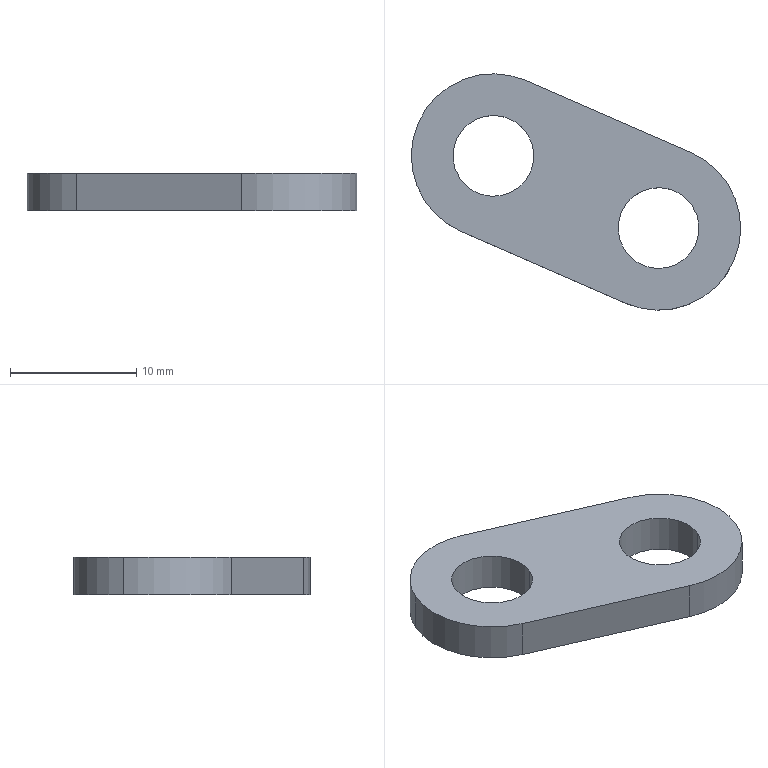Component | SolidWorks | CH-225-D-1_225-D-04-1 | 1 solid | 11 faces | box 26.08 x 18.71 x 3 mm | volume 762 mm3 | cylinder 7 | plane 4 | commonest cylinder face diameters 6.4 x4 13 x3
STEP:
#1=CARTESIAN_POINT('',(1.542,2.996,4.761));
#2=VERTEX_POINT('',#1);
#3=CARTESIAN_POINT('',(1.773,2.895,4.761));
#4=VERTEX_POINT('',#3);
#5=CARTESIAN_POINT('',(1.658,2.945,4.761));
#6=DIRECTION('',(0.,0.,1.));
#7=DIRECTION('',(-0.9164,0.4003,0.));
#8=AXIS2_PLACEMENT_3D('',#5,#6,#7);
#9=CIRCLE('',#8,0.126);
#10=EDGE_CURVE('',#2,#4,#9,.T.);
#11=ORIENTED_EDGE('',*,*,#10,.T.);
#12=CARTESIAN_POINT('',(1.773,2.895,4.643));
#13=VERTEX_POINT('',#12);
#14=CARTESIAN_POINT('',(1.773,2.895,4.761));
#15=DIRECTION('',(0.,0.,-1.));
#16=VECTOR('',#15,39.37);
#17=LINE('',#14,#16);
#18=EDGE_CURVE('',#4,#13,#17,.T.);
#19=ORIENTED_EDGE('',*,*,#18,.T.);
#20=CARTESIAN_POINT('',(1.542,2.996,4.643));
#21=VERTEX_POINT('',#20);
#22=CARTESIAN_POINT('',(1.658,2.945,4.643));
#23=DIRECTION('',(0.,0.,-1.));
#24=DIRECTION('',(-0.9164,0.4003,0.));
#25=AXIS2_PLACEMENT_3D('',#22,#23,#24);
#26=CIRCLE('',#25,0.126);
#27=EDGE_CURVE('',#13,#21,#26,.T.);
#28=ORIENTED_EDGE('',*,*,#27,.T.);
#29=CARTESIAN_POINT('',(1.542,2.996,4.761));
#30=DIRECTION('',(0.,0.,-1.));
#31=VECTOR('',#30,39.37);
#32=LINE('',#29,#31);
#33=EDGE_CURVE('',#2,#21,#32,.T.);
#34=ORIENTED_EDGE('',*,*,#33,.F.);
#35=EDGE_LOOP('',(#11,#19,#28,#34));
#36=FACE_OUTER_BOUND('',#35,.T.);
#37=CARTESIAN_POINT('',(1.658,2.945,4.761));
#38=DIRECTION('',(0.,0.,-1.));
#39=DIRECTION('',(-0.9164,0.4003,0.));
#40=AXIS2_PLACEMENT_3D('',#37,#38,#39);
#41=CYLINDRICAL_SURFACE('',#40,0.126);
#42=ADVANCED_FACE('',(#36),#41,.F.);
#43=CARTESIAN_POINT('',(2.288,2.67,4.761));
#44=VERTEX_POINT('',#43);
#45=CARTESIAN_POINT('',(2.057,2.771,4.761));
#46=VERTEX_POINT('',#45);
#47=CARTESIAN_POINT('',(2.172,2.721,4.761));
#48=DIRECTION('',(0.,0.,-1.));
#49=DIRECTION('',(-0.9164,0.4003,0.));
#50=AXIS2_PLACEMENT_3D('',#47,#48,#49);
#51=CIRCLE('',#50,0.126);
#52=EDGE_CURVE('',#44,#46,#51,.T.);
#53=ORIENTED_EDGE('',*,*,#52,.F.);
#54=CARTESIAN_POINT('',(2.288,2.67,4.643));
#55=VERTEX_POINT('',#54);
#56=CARTESIAN_POINT('',(2.288,2.67,4.761));
#57=DIRECTION('',(0.,0.,-1.));
#58=VECTOR('',#57,39.37);
#59=LINE('',#56,#58);
#60=EDGE_CURVE('',#44,#55,#59,.T.);
#61=ORIENTED_EDGE('',*,*,#60,.T.);
#62=CARTESIAN_POINT('',(2.057,2.771,4.643));
#63=VERTEX_POINT('',#62);
#64=CARTESIAN_POINT('',(2.172,2.721,4.643));
#65=DIRECTION('',(0.,0.,-1.));
#66=DIRECTION('',(-0.9164,0.4003,0.));
#67=AXIS2_PLACEMENT_3D('',#64,#65,#66);
#68=CIRCLE('',#67,0.126);
#69=EDGE_CURVE('',#55,#63,#68,.T.);
#70=ORIENTED_EDGE('',*,*,#69,.T.);
#71=CARTESIAN_POINT('',(2.057,2.771,4.761));
#72=DIRECTION('',(0.,0.,-1.));
#73=VECTOR('',#72,39.37);
#74=LINE('',#71,#73);
#75=EDGE_CURVE('',#46,#63,#74,.T.);
#76=ORIENTED_EDGE('',*,*,#75,.F.);
#77=EDGE_LOOP('',(#53,#61,#70,#76));
#78=FACE_OUTER_BOUND('',#77,.T.);
#79=CARTESIAN_POINT('',(2.172,2.721,4.761));
#80=DIRECTION('',(0.,0.,-1.));
#81=DIRECTION('',(-0.9164,0.4003,0.));
#82=AXIS2_PLACEMENT_3D('',#79,#80,#81);
#83=CYLINDRICAL_SURFACE('',#82,0.126);
#84=ADVANCED_FACE('',(#78),#83,.F.);
#85=CARTESIAN_POINT('',(1.423,3.048,4.761));
#86=VERTEX_POINT('',#85);
#87=CARTESIAN_POINT('',(1.555,2.711,4.761));
#88=VERTEX_POINT('',#87);
#89=CARTESIAN_POINT('',(1.658,2.945,4.761));
#90=DIRECTION('',(0.,0.,1.));
#91=DIRECTION('',(-0.9164,0.4003,0.));
#92=AXIS2_PLACEMENT_3D('',#89,#90,#91);
#93=CIRCLE('',#92,0.2559);
#94=EDGE_CURVE('',#86,#88,#93,.T.);
#95=ORIENTED_EDGE('',*,*,#94,.F.);
#96=CARTESIAN_POINT('',(1.423,3.048,4.643));
#97=VERTEX_POINT('',#96);
#98=CARTESIAN_POINT('',(1.423,3.048,4.761));
#99=DIRECTION('',(0.,0.,-1.));
#100=VECTOR('',#99,39.37);
#101=LINE('',#98,#100);
#102=EDGE_CURVE('',#86,#97,#101,.T.);
#103=ORIENTED_EDGE('',*,*,#102,.T.);
#104=CARTESIAN_POINT('',(1.555,2.711,4.643));
#105=VERTEX_POINT('',#104);
#106=CARTESIAN_POINT('',(1.658,2.945,4.643));
#107=DIRECTION('',(0.,0.,1.));
#108=DIRECTION('',(-0.9164,0.4003,0.));
#109=AXIS2_PLACEMENT_3D('',#106,#107,#108);
#110=CIRCLE('',#109,0.2559);
#111=EDGE_CURVE('',#97,#105,#110,.T.);
#112=ORIENTED_EDGE('',*,*,#111,.T.);
#113=CARTESIAN_POINT('',(1.555,2.711,4.702));
#114=DIRECTION('',(0.,0.,1.));
#115=VECTOR('',#114,39.37);
#116=LINE('',#113,#115);
#117=EDGE_CURVE('',#105,#88,#116,.T.);
#118=ORIENTED_EDGE('',*,*,#117,.T.);
#119=EDGE_LOOP('',(#95,#103,#112,#118));
#120=FACE_OUTER_BOUND('',#119,.T.);
#121=CARTESIAN_POINT('',(1.658,2.945,4.761));
#122=DIRECTION('',(0.,0.,-1.));
#123=DIRECTION('',(-0.9164,0.4003,0.));
#124=AXIS2_PLACEMENT_3D('',#121,#122,#123);
#125=CYLINDRICAL_SURFACE('',#124,0.2559);
#126=ADVANCED_FACE('',(#120),#125,.T.);
#127=ORIENTED_EDGE('',*,*,#18,.F.);
#128=CARTESIAN_POINT('',(1.658,2.945,4.761));
#129=DIRECTION('',(0.,0.,1.));
#130=DIRECTION('',(-0.9164,0.4003,0.));
#131=AXIS2_PLACEMENT_3D('',#128,#129,#130);
#132=CIRCLE('',#131,0.126);
#133=EDGE_CURVE('',#4,#2,#132,.T.);
#134=ORIENTED_EDGE('',*,*,#133,.T.);
#135=ORIENTED_EDGE('',*,*,#33,.T.);
#136=CARTESIAN_POINT('',(1.658,2.945,4.643));
#137=DIRECTION('',(0.,0.,-1.));
#138=DIRECTION('',(-0.9164,0.4003,0.));
#139=AXIS2_PLACEMENT_3D('',#136,#137,#138);
#140=CIRCLE('',#139,0.126);
#141=EDGE_CURVE('',#21,#13,#140,.T.);
#142=ORIENTED_EDGE('',*,*,#141,.T.);
#143=EDGE_LOOP('',(#127,#134,#135,#142));
#144=FACE_OUTER_BOUND('',#143,.T.);
#145=CARTESIAN_POINT('',(1.658,2.945,4.761));
#146=DIRECTION('',(0.,0.,-1.));
#147=DIRECTION('',(-0.9164,0.4003,0.));
#148=AXIS2_PLACEMENT_3D('',#145,#146,#147);
#149=CYLINDRICAL_SURFACE('',#148,0.126);
#150=ADVANCED_FACE('',(#144),#149,.F.);
#151=ORIENTED_EDGE('',*,*,#141,.F.);
#152=ORIENTED_EDGE('',*,*,#27,.F.);
#153=EDGE_LOOP('',(#151,#152));
#154=FACE_BOUND('',#153,.T.);
#155=CARTESIAN_POINT('',(2.172,2.721,4.643));
#156=DIRECTION('',(0.,0.,-1.));
#157=DIRECTION('',(-0.9164,0.4003,0.));
#158=AXIS2_PLACEMENT_3D('',#155,#156,#157);
#159=CIRCLE('',#158,0.126);
#160=EDGE_CURVE('',#63,#55,#159,.T.);
#161=ORIENTED_EDGE('',*,*,#160,.F.);
#162=ORIENTED_EDGE('',*,*,#69,.F.);
#163=EDGE_LOOP('',(#161,#162));
#164=FACE_BOUND('',#163,.T.);
#165=CARTESIAN_POINT('',(2.275,2.955,4.643));
#166=VERTEX_POINT('',#165);
#167=CARTESIAN_POINT('',(1.76,3.18,4.643));
#168=VERTEX_POINT('',#167);
#169=CARTESIAN_POINT('',(2.017,3.067,4.643));
#170=DIRECTION('',(-0.9164,0.4003,0.));
#171=VECTOR('',#170,39.37);
#172=LINE('',#169,#171);
#173=EDGE_CURVE('',#166,#168,#172,.T.);
#174=ORIENTED_EDGE('',*,*,#173,.F.);
#175=CARTESIAN_POINT('',(2.07,2.486,4.643));
#176=VERTEX_POINT('',#175);
#177=CARTESIAN_POINT('',(2.172,2.721,4.643));
#178=DIRECTION('',(0.,0.,1.));
#179=DIRECTION('',(-0.9164,0.4003,0.));
#180=AXIS2_PLACEMENT_3D('',#177,#178,#179);
#181=CIRCLE('',#180,0.2559);
#182=EDGE_CURVE('',#176,#166,#181,.T.);
#183=ORIENTED_EDGE('',*,*,#182,.F.);
#184=CARTESIAN_POINT('',(1.813,2.598,4.643));
#185=DIRECTION('',(0.9164,-0.4003,0.));
#186=VECTOR('',#185,39.37);
#187=LINE('',#184,#186);
#188=EDGE_CURVE('',#105,#176,#187,.T.);
#189=ORIENTED_EDGE('',*,*,#188,.F.);
#190=ORIENTED_EDGE('',*,*,#111,.F.);
#191=CARTESIAN_POINT('',(1.658,2.945,4.643));
#192=DIRECTION('',(0.,0.,1.));
#193=DIRECTION('',(-0.9164,0.4003,0.));
#194=AXIS2_PLACEMENT_3D('',#191,#192,#193);
#195=CIRCLE('',#194,0.2559);
#196=EDGE_CURVE('',#168,#97,#195,.T.);
#197=ORIENTED_EDGE('',*,*,#196,.F.);
#198=EDGE_LOOP('',(#174,#183,#189,#190,#197));
#199=FACE_OUTER_BOUND('',#198,.T.);
#200=CARTESIAN_POINT('',(1.315,2.816,4.643));
#201=DIRECTION('',(0.,0.,1.));
#202=DIRECTION('',(0.9164,-0.4003,0.));
#203=AXIS2_PLACEMENT_3D('',#200,#201,#202);
#204=PLANE('',#203);
#205=ADVANCED_FACE('',(#154,#164,#199),#204,.F.);
#206=ORIENTED_EDGE('',*,*,#10,.F.);
#207=ORIENTED_EDGE('',*,*,#133,.F.);
#208=EDGE_LOOP('',(#206,#207));
#209=FACE_BOUND('',#208,.T.);
#210=CARTESIAN_POINT('',(2.172,2.721,4.761));
#211=DIRECTION('',(0.,0.,-1.));
#212=DIRECTION('',(-0.9164,0.4003,0.));
#213=AXIS2_PLACEMENT_3D('',#210,#211,#212);
#214=CIRCLE('',#213,0.126);
#215=EDGE_CURVE('',#46,#44,#214,.T.);
#216=ORIENTED_EDGE('',*,*,#215,.T.);
#217=ORIENTED_EDGE('',*,*,#52,.T.);
#218=EDGE_LOOP('',(#216,#217));
#219=FACE_BOUND('',#218,.T.);
#220=CARTESIAN_POINT('',(2.07,2.486,4.761));
#221=VERTEX_POINT('',#220);
#222=CARTESIAN_POINT('',(2.275,2.955,4.761));
#223=VERTEX_POINT('',#222);
#224=CARTESIAN_POINT('',(2.172,2.721,4.761));
#225=DIRECTION('',(0.,0.,1.));
#226=DIRECTION('',(-0.9164,0.4003,0.));
#227=AXIS2_PLACEMENT_3D('',#224,#225,#226);
#228=CIRCLE('',#227,0.2559);
#229=EDGE_CURVE('',#221,#223,#228,.T.);
#230=ORIENTED_EDGE('',*,*,#229,.T.);
#231=CARTESIAN_POINT('',(1.76,3.18,4.761));
#232=VERTEX_POINT('',#231);
#233=CARTESIAN_POINT('',(2.017,3.067,4.761));
#234=DIRECTION('',(-0.9164,0.4003,0.));
#235=VECTOR('',#234,39.37);
#236=LINE('',#233,#235);
#237=EDGE_CURVE('',#223,#232,#236,.T.);
#238=ORIENTED_EDGE('',*,*,#237,.T.);
#239=CARTESIAN_POINT('',(1.658,2.945,4.761));
#240=DIRECTION('',(0.,0.,1.));
#241=DIRECTION('',(-0.9164,0.4003,0.));
#242=AXIS2_PLACEMENT_3D('',#239,#240,#241);
#243=CIRCLE('',#242,0.2559);
#244=EDGE_CURVE('',#232,#86,#243,.T.);
#245=ORIENTED_EDGE('',*,*,#244,.T.);
#246=ORIENTED_EDGE('',*,*,#94,.T.);
#247=CARTESIAN_POINT('',(1.813,2.598,4.761));
#248=DIRECTION('',(0.9164,-0.4003,0.));
#249=VECTOR('',#248,39.37);
#250=LINE('',#247,#249);
#251=EDGE_CURVE('',#88,#221,#250,.T.);
#252=ORIENTED_EDGE('',*,*,#251,.T.);
#253=EDGE_LOOP('',(#230,#238,#245,#246,#252));
#254=FACE_OUTER_BOUND('',#253,.T.);
#255=CARTESIAN_POINT('',(1.315,2.816,4.761));
#256=DIRECTION('',(0.,0.,1.));
#257=DIRECTION('',(0.9164,-0.4003,0.));
#258=AXIS2_PLACEMENT_3D('',#255,#256,#257);
#259=PLANE('',#258);
#260=ADVANCED_FACE('',(#209,#219,#254),#259,.T.);
#261=ORIENTED_EDGE('',*,*,#60,.F.);
#262=ORIENTED_EDGE('',*,*,#215,.F.);
#263=ORIENTED_EDGE('',*,*,#75,.T.);
#264=ORIENTED_EDGE('',*,*,#160,.T.);
#265=EDGE_LOOP('',(#261,#262,#263,#264));
#266=FACE_OUTER_BOUND('',#265,.T.);
#267=CARTESIAN_POINT('',(2.172,2.721,4.761));
#268=DIRECTION('',(0.,0.,-1.));
#269=DIRECTION('',(-0.9164,0.4003,0.));
#270=AXIS2_PLACEMENT_3D('',#267,#268,#269);
#271=CYLINDRICAL_SURFACE('',#270,0.126);
#272=ADVANCED_FACE('',(#266),#271,.F.);
#273=ORIENTED_EDGE('',*,*,#102,.F.);
#274=ORIENTED_EDGE('',*,*,#244,.F.);
#275=CARTESIAN_POINT('',(1.76,3.18,4.702));
#276=DIRECTION('',(0.,0.,1.));
#277=VECTOR('',#276,39.37);
#278=LINE('',#275,#277);
#279=EDGE_CURVE('',#168,#232,#278,.T.);
#280=ORIENTED_EDGE('',*,*,#279,.F.);
#281=ORIENTED_EDGE('',*,*,#196,.T.);
#282=EDGE_LOOP('',(#273,#274,#280,#281));
#283=FACE_OUTER_BOUND('',#282,.T.);
#284=CARTESIAN_POINT('',(1.658,2.945,4.761));
#285=DIRECTION('',(0.,0.,-1.));
#286=DIRECTION('',(-0.9164,0.4003,0.));
#287=AXIS2_PLACEMENT_3D('',#284,#285,#286);
#288=CYLINDRICAL_SURFACE('',#287,0.2559);
#289=ADVANCED_FACE('',(#283),#288,.T.);
#290=ORIENTED_EDGE('',*,*,#279,.T.);
#291=ORIENTED_EDGE('',*,*,#237,.F.);
#292=CARTESIAN_POINT('',(2.275,2.955,4.702));
#293=DIRECTION('',(0.,0.,1.));
#294=VECTOR('',#293,39.37);
#295=LINE('',#292,#294);
#296=EDGE_CURVE('',#166,#223,#295,.T.);
#297=ORIENTED_EDGE('',*,*,#296,.F.);
#298=ORIENTED_EDGE('',*,*,#173,.T.);
#299=EDGE_LOOP('',(#290,#291,#297,#298));
#300=FACE_OUTER_BOUND('',#299,.T.);
#301=CARTESIAN_POINT('',(1.76,3.18,4.643));
#302=DIRECTION('',(-0.4003,-0.9164,0.));
#303=DIRECTION('',(0.9164,-0.4003,0.));
#304=AXIS2_PLACEMENT_3D('',#301,#302,#303);
#305=PLANE('',#304);
#306=ADVANCED_FACE('',(#300),#305,.F.);
#307=ORIENTED_EDGE('',*,*,#296,.T.);
#308=ORIENTED_EDGE('',*,*,#229,.F.);
#309=CARTESIAN_POINT('',(2.07,2.486,4.702));
#310=DIRECTION('',(0.,0.,1.));
#311=VECTOR('',#310,39.37);
#312=LINE('',#309,#311);
#313=EDGE_CURVE('',#176,#221,#312,.T.);
#314=ORIENTED_EDGE('',*,*,#313,.F.);
#315=ORIENTED_EDGE('',*,*,#182,.T.);
#316=EDGE_LOOP('',(#307,#308,#314,#315));
#317=FACE_OUTER_BOUND('',#316,.T.);
#318=CARTESIAN_POINT('',(2.172,2.721,4.761));
#319=DIRECTION('',(0.,0.,-1.));
#320=DIRECTION('',(-0.9164,0.4003,0.));
#321=AXIS2_PLACEMENT_3D('',#318,#319,#320);
#322=CYLINDRICAL_SURFACE('',#321,0.2559);
#323=ADVANCED_FACE('',(#317),#322,.T.);
#324=ORIENTED_EDGE('',*,*,#313,.T.);
#325=ORIENTED_EDGE('',*,*,#251,.F.);
#326=ORIENTED_EDGE('',*,*,#117,.F.);
#327=ORIENTED_EDGE('',*,*,#188,.T.);
#328=EDGE_LOOP('',(#324,#325,#326,#327));
#329=FACE_OUTER_BOUND('',#328,.T.);
#330=CARTESIAN_POINT('',(2.07,2.486,4.643));
#331=DIRECTION('',(0.4003,0.9164,0.));
#332=DIRECTION('',(-0.9164,0.4003,0.));
#333=AXIS2_PLACEMENT_3D('',#330,#331,#332);
#334=PLANE('',#333);
#335=ADVANCED_FACE('',(#329),#334,.F.);
#336=CLOSED_SHELL('',(#42,#84,#126,#150,#205,#260,#272,#289,#306,#323,#335));
#337=MANIFOLD_SOLID_BREP('',#336);
#338=CARTESIAN_POINT('',(0.,0.,0.));
#339=DIRECTION('',(0.,0.,1.));
#340=DIRECTION('',(1.,0.,0.));
#341=AXIS2_PLACEMENT_3D('',#338,#339,#340);
#342=(LENGTH_UNIT()NAMED_UNIT(*)SI_UNIT($,.METRE.));
#343=LENGTH_MEASURE_WITH_UNIT(LENGTH_MEASURE(0.0254),#342);
#344=DIMENSIONAL_EXPONENTS(1.,0.,0.,0.,0.,0.,0.);
#345=(CONVERSION_BASED_UNIT('',#343)LENGTH_UNIT()NAMED_UNIT(#344));
#346=UNCERTAINTY_MEASURE_WITH_UNIT(LENGTH_MEASURE(0.00001),#345,'','');
#347=(NAMED_UNIT(*)PLANE_ANGLE_UNIT()SI_UNIT($,.RADIAN.));
#348=(NAMED_UNIT(*)SI_UNIT($,.STERADIAN.)SOLID_ANGLE_UNIT());
#349=(GEOMETRIC_REPRESENTATION_CONTEXT(3)GLOBAL_UNCERTAINTY_ASSIGNED_CONTEXT((#346))GLOBAL_UNIT_ASSIGNED_CONTEXT((#345,#347,#348))REPRESENTATION_CONTEXT('',''));
#350=ADVANCED_BREP_SHAPE_REPRESENTATION('',(#337,#341),#349);
#351=COLOUR_RGB('',0.7922,0.8196,0.9333);
#352=FILL_AREA_STYLE_COLOUR('',#351);
#353=FILL_AREA_STYLE('',(#352));
#354=SURFACE_STYLE_FILL_AREA(#353);
#355=SURFACE_SIDE_STYLE('',(#354));
#356=SURFACE_STYLE_USAGE(.BOTH.,#355);
#357=PRESENTATION_STYLE_ASSIGNMENT((#356));
#358=STYLED_ITEM('',(#357),#337);
#359=PRESENTATION_LAYER_ASSIGNMENT('','',(#358));
#360=(LENGTH_UNIT()NAMED_UNIT(*)SI_UNIT($,.METRE.));
#361=LENGTH_MEASURE_WITH_UNIT(LENGTH_MEASURE(0.0254),#360);
#362=DIMENSIONAL_EXPONENTS(1.,0.,0.,0.,0.,0.,0.);
#363=(CONVERSION_BASED_UNIT('',#361)LENGTH_UNIT()NAMED_UNIT(#362));
#364=UNCERTAINTY_MEASURE_WITH_UNIT(LENGTH_MEASURE(0.00001),#363,'','');
#365=(NAMED_UNIT(*)PLANE_ANGLE_UNIT()SI_UNIT($,.RADIAN.));
#366=(NAMED_UNIT(*)SI_UNIT($,.STERADIAN.)SOLID_ANGLE_UNIT());
#367=(GEOMETRIC_REPRESENTATION_CONTEXT(3)GLOBAL_UNCERTAINTY_ASSIGNED_CONTEXT((#364))GLOBAL_UNIT_ASSIGNED_CONTEXT((#363,#365,#366))REPRESENTATION_CONTEXT('',''));
#368=MECHANICAL_DESIGN_GEOMETRIC_PRESENTATION_REPRESENTATION('',(#358),#367);